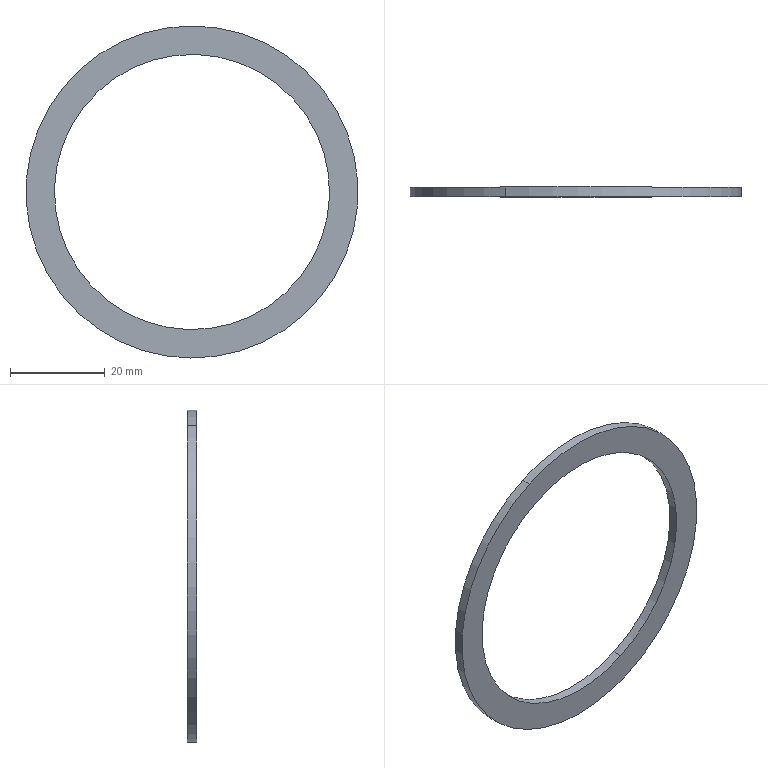Component | SolidWorks | Assembly4.1-1_117.1-1 | 1 solid | 6 faces | box 70 x 2 x 70 mm | volume 2413 mm3 | cylinder 4 | plane 2 | commonest cylinder face diameters 58 x2 70 x2
build123d program:
from build123d import *

# Parameters (mm, degrees)
SKETCH1_R           = 35
SKETCH1_R_2         = 29
BOSS_EXTRUDE1_DEPTH = 2


with BuildPart() as part:
    # Sketch1 → Boss-Extrude1 (new body)
    with BuildSketch(Plane.XY):
        Circle(SKETCH1_R)
        Circle(SKETCH1_R_2, mode=Mode.SUBTRACT)
    extrude(amount=BOSS_EXTRUDE1_DEPTH)


solid = part.part

# Placed as in the assembly
solid = solid.moved(Location((0, -29.5, -0.4), (90, 0, 0)))
STEP:
#1=COLOUR_RGB('',0.7922,0.8196,0.9333);
#2=FILL_AREA_STYLE_COLOUR('',#1);
#3=FILL_AREA_STYLE('',(#2));
#4=SURFACE_STYLE_FILL_AREA(#3);
#5=SURFACE_SIDE_STYLE('',(#4));
#6=SURFACE_STYLE_USAGE(.BOTH.,#5);
#7=PRESENTATION_STYLE_ASSIGNMENT((#6));
#8=CARTESIAN_POINT('',(0.4853,-1.24,-1.049));
#9=VERTEX_POINT('',#8);
#10=CARTESIAN_POINT('',(-0.4853,-1.24,1.018));
#11=VERTEX_POINT('',#10);
#12=CARTESIAN_POINT('',(-0.,-1.24,-0.01575));
#13=DIRECTION('',(-0.,-1.,0.));
#14=DIRECTION('',(-0.4251,0.,0.9052));
#15=AXIS2_PLACEMENT_3D('',#12,#13,#14);
#16=CIRCLE('',#15,1.142);
#17=EDGE_CURVE('',#9,#11,#16,.T.);
#18=ORIENTED_EDGE('',*,*,#17,.T.);
#19=CARTESIAN_POINT('',(-0.4853,-1.161,1.018));
#20=VERTEX_POINT('',#19);
#21=CARTESIAN_POINT('',(-0.4853,-1.24,1.018));
#22=DIRECTION('',(0.,1.,-0.));
#23=VECTOR('',#22,39.37);
#24=LINE('',#21,#23);
#25=EDGE_CURVE('',#11,#20,#24,.T.);
#26=ORIENTED_EDGE('',*,*,#25,.T.);
#27=CARTESIAN_POINT('',(0.4853,-1.161,-1.049));
#28=VERTEX_POINT('',#27);
#29=CARTESIAN_POINT('',(-0.,-1.161,-0.01575));
#30=DIRECTION('',(-0.,-1.,0.));
#31=DIRECTION('',(-0.4251,0.,0.9052));
#32=AXIS2_PLACEMENT_3D('',#29,#30,#31);
#33=CIRCLE('',#32,1.142);
#34=EDGE_CURVE('',#28,#20,#33,.T.);
#35=ORIENTED_EDGE('',*,*,#34,.F.);
#36=CARTESIAN_POINT('',(0.4853,-1.24,-1.049));
#37=DIRECTION('',(0.,1.,-0.));
#38=VECTOR('',#37,39.37);
#39=LINE('',#36,#38);
#40=EDGE_CURVE('',#9,#28,#39,.T.);
#41=ORIENTED_EDGE('',*,*,#40,.F.);
#42=EDGE_LOOP('',(#18,#26,#35,#41));
#43=FACE_OUTER_BOUND('',#42,.T.);
#44=CARTESIAN_POINT('',(-0.,-1.24,-0.01575));
#45=DIRECTION('',(0.,1.,-0.));
#46=DIRECTION('',(0.4251,0.,-0.9052));
#47=AXIS2_PLACEMENT_3D('',#44,#45,#46);
#48=CYLINDRICAL_SURFACE('',#47,1.142);
#49=ADVANCED_FACE('',(#43),#48,.F.);
#50=CARTESIAN_POINT('',(-0.5857,-1.24,1.232));
#51=VERTEX_POINT('',#50);
#52=CARTESIAN_POINT('',(0.5857,-1.24,-1.263));
#53=VERTEX_POINT('',#52);
#54=CARTESIAN_POINT('',(-0.,-1.24,-0.01575));
#55=DIRECTION('',(-0.,-1.,0.));
#56=DIRECTION('',(-0.4251,0.,0.9052));
#57=AXIS2_PLACEMENT_3D('',#54,#55,#56);
#58=CIRCLE('',#57,1.378);
#59=EDGE_CURVE('',#51,#53,#58,.T.);
#60=ORIENTED_EDGE('',*,*,#59,.F.);
#61=CARTESIAN_POINT('',(-0.5857,-1.161,1.232));
#62=VERTEX_POINT('',#61);
#63=CARTESIAN_POINT('',(-0.5857,-1.24,1.232));
#64=DIRECTION('',(0.,1.,-0.));
#65=VECTOR('',#64,39.37);
#66=LINE('',#63,#65);
#67=EDGE_CURVE('',#51,#62,#66,.T.);
#68=ORIENTED_EDGE('',*,*,#67,.T.);
#69=CARTESIAN_POINT('',(0.5857,-1.161,-1.263));
#70=VERTEX_POINT('',#69);
#71=CARTESIAN_POINT('',(-0.,-1.161,-0.01575));
#72=DIRECTION('',(-0.,-1.,0.));
#73=DIRECTION('',(-0.4251,0.,0.9052));
#74=AXIS2_PLACEMENT_3D('',#71,#72,#73);
#75=CIRCLE('',#74,1.378);
#76=EDGE_CURVE('',#62,#70,#75,.T.);
#77=ORIENTED_EDGE('',*,*,#76,.T.);
#78=CARTESIAN_POINT('',(0.5857,-1.24,-1.263));
#79=DIRECTION('',(0.,1.,-0.));
#80=VECTOR('',#79,39.37);
#81=LINE('',#78,#80);
#82=EDGE_CURVE('',#53,#70,#81,.T.);
#83=ORIENTED_EDGE('',*,*,#82,.F.);
#84=EDGE_LOOP('',(#60,#68,#77,#83));
#85=FACE_OUTER_BOUND('',#84,.T.);
#86=CARTESIAN_POINT('',(-0.,-1.24,-0.01575));
#87=DIRECTION('',(0.,1.,-0.));
#88=DIRECTION('',(0.4251,0.,-0.9052));
#89=AXIS2_PLACEMENT_3D('',#86,#87,#88);
#90=CYLINDRICAL_SURFACE('',#89,1.378);
#91=ADVANCED_FACE('',(#85),#90,.T.);
#92=CARTESIAN_POINT('',(-0.,-1.24,-0.01575));
#93=DIRECTION('',(-0.,-1.,0.));
#94=DIRECTION('',(-0.4251,0.,0.9052));
#95=AXIS2_PLACEMENT_3D('',#92,#93,#94);
#96=CIRCLE('',#95,1.378);
#97=EDGE_CURVE('',#53,#51,#96,.T.);
#98=ORIENTED_EDGE('',*,*,#97,.T.);
#99=ORIENTED_EDGE('',*,*,#59,.T.);
#100=EDGE_LOOP('',(#98,#99));
#101=FACE_OUTER_BOUND('',#100,.T.);
#102=ORIENTED_EDGE('',*,*,#17,.F.);
#103=CARTESIAN_POINT('',(-0.,-1.24,-0.01575));
#104=DIRECTION('',(-0.,-1.,0.));
#105=DIRECTION('',(-0.4251,0.,0.9052));
#106=AXIS2_PLACEMENT_3D('',#103,#104,#105);
#107=CIRCLE('',#106,1.142);
#108=EDGE_CURVE('',#11,#9,#107,.T.);
#109=ORIENTED_EDGE('',*,*,#108,.F.);
#110=EDGE_LOOP('',(#102,#109));
#111=FACE_BOUND('',#110,.T.);
#112=CARTESIAN_POINT('',(-0.,-1.24,-0.01575));
#113=DIRECTION('',(-0.,-1.,0.));
#114=DIRECTION('',(-0.4251,0.,0.9052));
#115=AXIS2_PLACEMENT_3D('',#112,#113,#114);
#116=PLANE('',#115);
#117=ADVANCED_FACE('',(#101,#111),#116,.T.);
#118=CARTESIAN_POINT('',(-0.,-1.161,-0.01575));
#119=DIRECTION('',(-0.,-1.,0.));
#120=DIRECTION('',(-0.4251,0.,0.9052));
#121=AXIS2_PLACEMENT_3D('',#118,#119,#120);
#122=CIRCLE('',#121,1.378);
#123=EDGE_CURVE('',#70,#62,#122,.T.);
#124=ORIENTED_EDGE('',*,*,#123,.F.);
#125=ORIENTED_EDGE('',*,*,#76,.F.);
#126=EDGE_LOOP('',(#124,#125));
#127=FACE_OUTER_BOUND('',#126,.T.);
#128=ORIENTED_EDGE('',*,*,#34,.T.);
#129=CARTESIAN_POINT('',(-0.,-1.161,-0.01575));
#130=DIRECTION('',(-0.,-1.,0.));
#131=DIRECTION('',(-0.4251,0.,0.9052));
#132=AXIS2_PLACEMENT_3D('',#129,#130,#131);
#133=CIRCLE('',#132,1.142);
#134=EDGE_CURVE('',#20,#28,#133,.T.);
#135=ORIENTED_EDGE('',*,*,#134,.T.);
#136=EDGE_LOOP('',(#128,#135));
#137=FACE_BOUND('',#136,.T.);
#138=CARTESIAN_POINT('',(-0.,-1.161,-0.01575));
#139=DIRECTION('',(-0.,-1.,0.));
#140=DIRECTION('',(-0.4251,0.,0.9052));
#141=AXIS2_PLACEMENT_3D('',#138,#139,#140);
#142=PLANE('',#141);
#143=ADVANCED_FACE('',(#127,#137),#142,.F.);
#144=ORIENTED_EDGE('',*,*,#67,.F.);
#145=ORIENTED_EDGE('',*,*,#97,.F.);
#146=ORIENTED_EDGE('',*,*,#82,.T.);
#147=ORIENTED_EDGE('',*,*,#123,.T.);
#148=EDGE_LOOP('',(#144,#145,#146,#147));
#149=FACE_OUTER_BOUND('',#148,.T.);
#150=CARTESIAN_POINT('',(-0.,-1.24,-0.01575));
#151=DIRECTION('',(0.,1.,-0.));
#152=DIRECTION('',(0.4251,0.,-0.9052));
#153=AXIS2_PLACEMENT_3D('',#150,#151,#152);
#154=CYLINDRICAL_SURFACE('',#153,1.378);
#155=ADVANCED_FACE('',(#149),#154,.T.);
#156=ORIENTED_EDGE('',*,*,#25,.F.);
#157=ORIENTED_EDGE('',*,*,#108,.T.);
#158=ORIENTED_EDGE('',*,*,#40,.T.);
#159=ORIENTED_EDGE('',*,*,#134,.F.);
#160=EDGE_LOOP('',(#156,#157,#158,#159));
#161=FACE_OUTER_BOUND('',#160,.T.);
#162=CARTESIAN_POINT('',(-0.,-1.24,-0.01575));
#163=DIRECTION('',(0.,1.,-0.));
#164=DIRECTION('',(0.4251,0.,-0.9052));
#165=AXIS2_PLACEMENT_3D('',#162,#163,#164);
#166=CYLINDRICAL_SURFACE('',#165,1.142);
#167=ADVANCED_FACE('',(#161),#166,.F.);
#168=CLOSED_SHELL('',(#49,#91,#117,#143,#155,#167));
#169=MANIFOLD_SOLID_BREP('',#168);
#170=STYLED_ITEM('',(#7),#169);
#171=(LENGTH_UNIT()NAMED_UNIT(*)SI_UNIT($,.METRE.));
#172=LENGTH_MEASURE_WITH_UNIT(LENGTH_MEASURE(0.0254),#171);
#173=DIMENSIONAL_EXPONENTS(1.,0.,0.,0.,0.,0.,0.);
#174=(CONVERSION_BASED_UNIT('',#172)LENGTH_UNIT()NAMED_UNIT(#173));
#175=UNCERTAINTY_MEASURE_WITH_UNIT(LENGTH_MEASURE(0.00001),#174,'','');
#176=(NAMED_UNIT(*)PLANE_ANGLE_UNIT()SI_UNIT($,.RADIAN.));
#177=(NAMED_UNIT(*)SI_UNIT($,.STERADIAN.)SOLID_ANGLE_UNIT());
#178=(GEOMETRIC_REPRESENTATION_CONTEXT(3)GLOBAL_UNCERTAINTY_ASSIGNED_CONTEXT((#175))GLOBAL_UNIT_ASSIGNED_CONTEXT((#174,#176,#177))REPRESENTATION_CONTEXT('',''));
#179=MECHANICAL_DESIGN_GEOMETRIC_PRESENTATION_REPRESENTATION('',(#170),#178);
#180=PRESENTATION_LAYER_ASSIGNMENT('','',(#170));
#181=CARTESIAN_POINT('',(0.,0.,0.));
#182=DIRECTION('',(0.,0.,1.));
#183=DIRECTION('',(1.,0.,0.));
#184=AXIS2_PLACEMENT_3D('',#181,#182,#183);
#185=(LENGTH_UNIT()NAMED_UNIT(*)SI_UNIT($,.METRE.));
#186=LENGTH_MEASURE_WITH_UNIT(LENGTH_MEASURE(0.0254),#185);
#187=DIMENSIONAL_EXPONENTS(1.,0.,0.,0.,0.,0.,0.);
#188=(CONVERSION_BASED_UNIT('',#186)LENGTH_UNIT()NAMED_UNIT(#187));
#189=UNCERTAINTY_MEASURE_WITH_UNIT(LENGTH_MEASURE(0.00001),#188,'','');
#190=(NAMED_UNIT(*)PLANE_ANGLE_UNIT()SI_UNIT($,.RADIAN.));
#191=(NAMED_UNIT(*)SI_UNIT($,.STERADIAN.)SOLID_ANGLE_UNIT());
#192=(GEOMETRIC_REPRESENTATION_CONTEXT(3)GLOBAL_UNCERTAINTY_ASSIGNED_CONTEXT((#189))GLOBAL_UNIT_ASSIGNED_CONTEXT((#188,#190,#191))REPRESENTATION_CONTEXT('',''));
#193=ADVANCED_BREP_SHAPE_REPRESENTATION('',(#169,#184),#192);